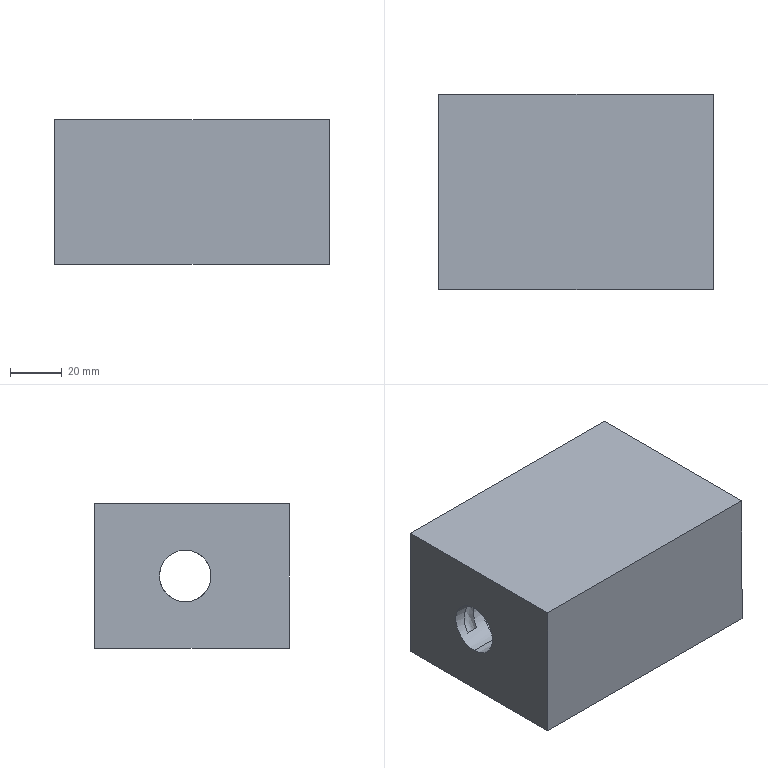Component | SolidWorks | NutSeat-1 | 1 solid | 41 faces | volume 404184 mm3 | cylinder 29 | plane 11 | spline 1 | commonest cylinder face diameters 20 x21 4.542 x8